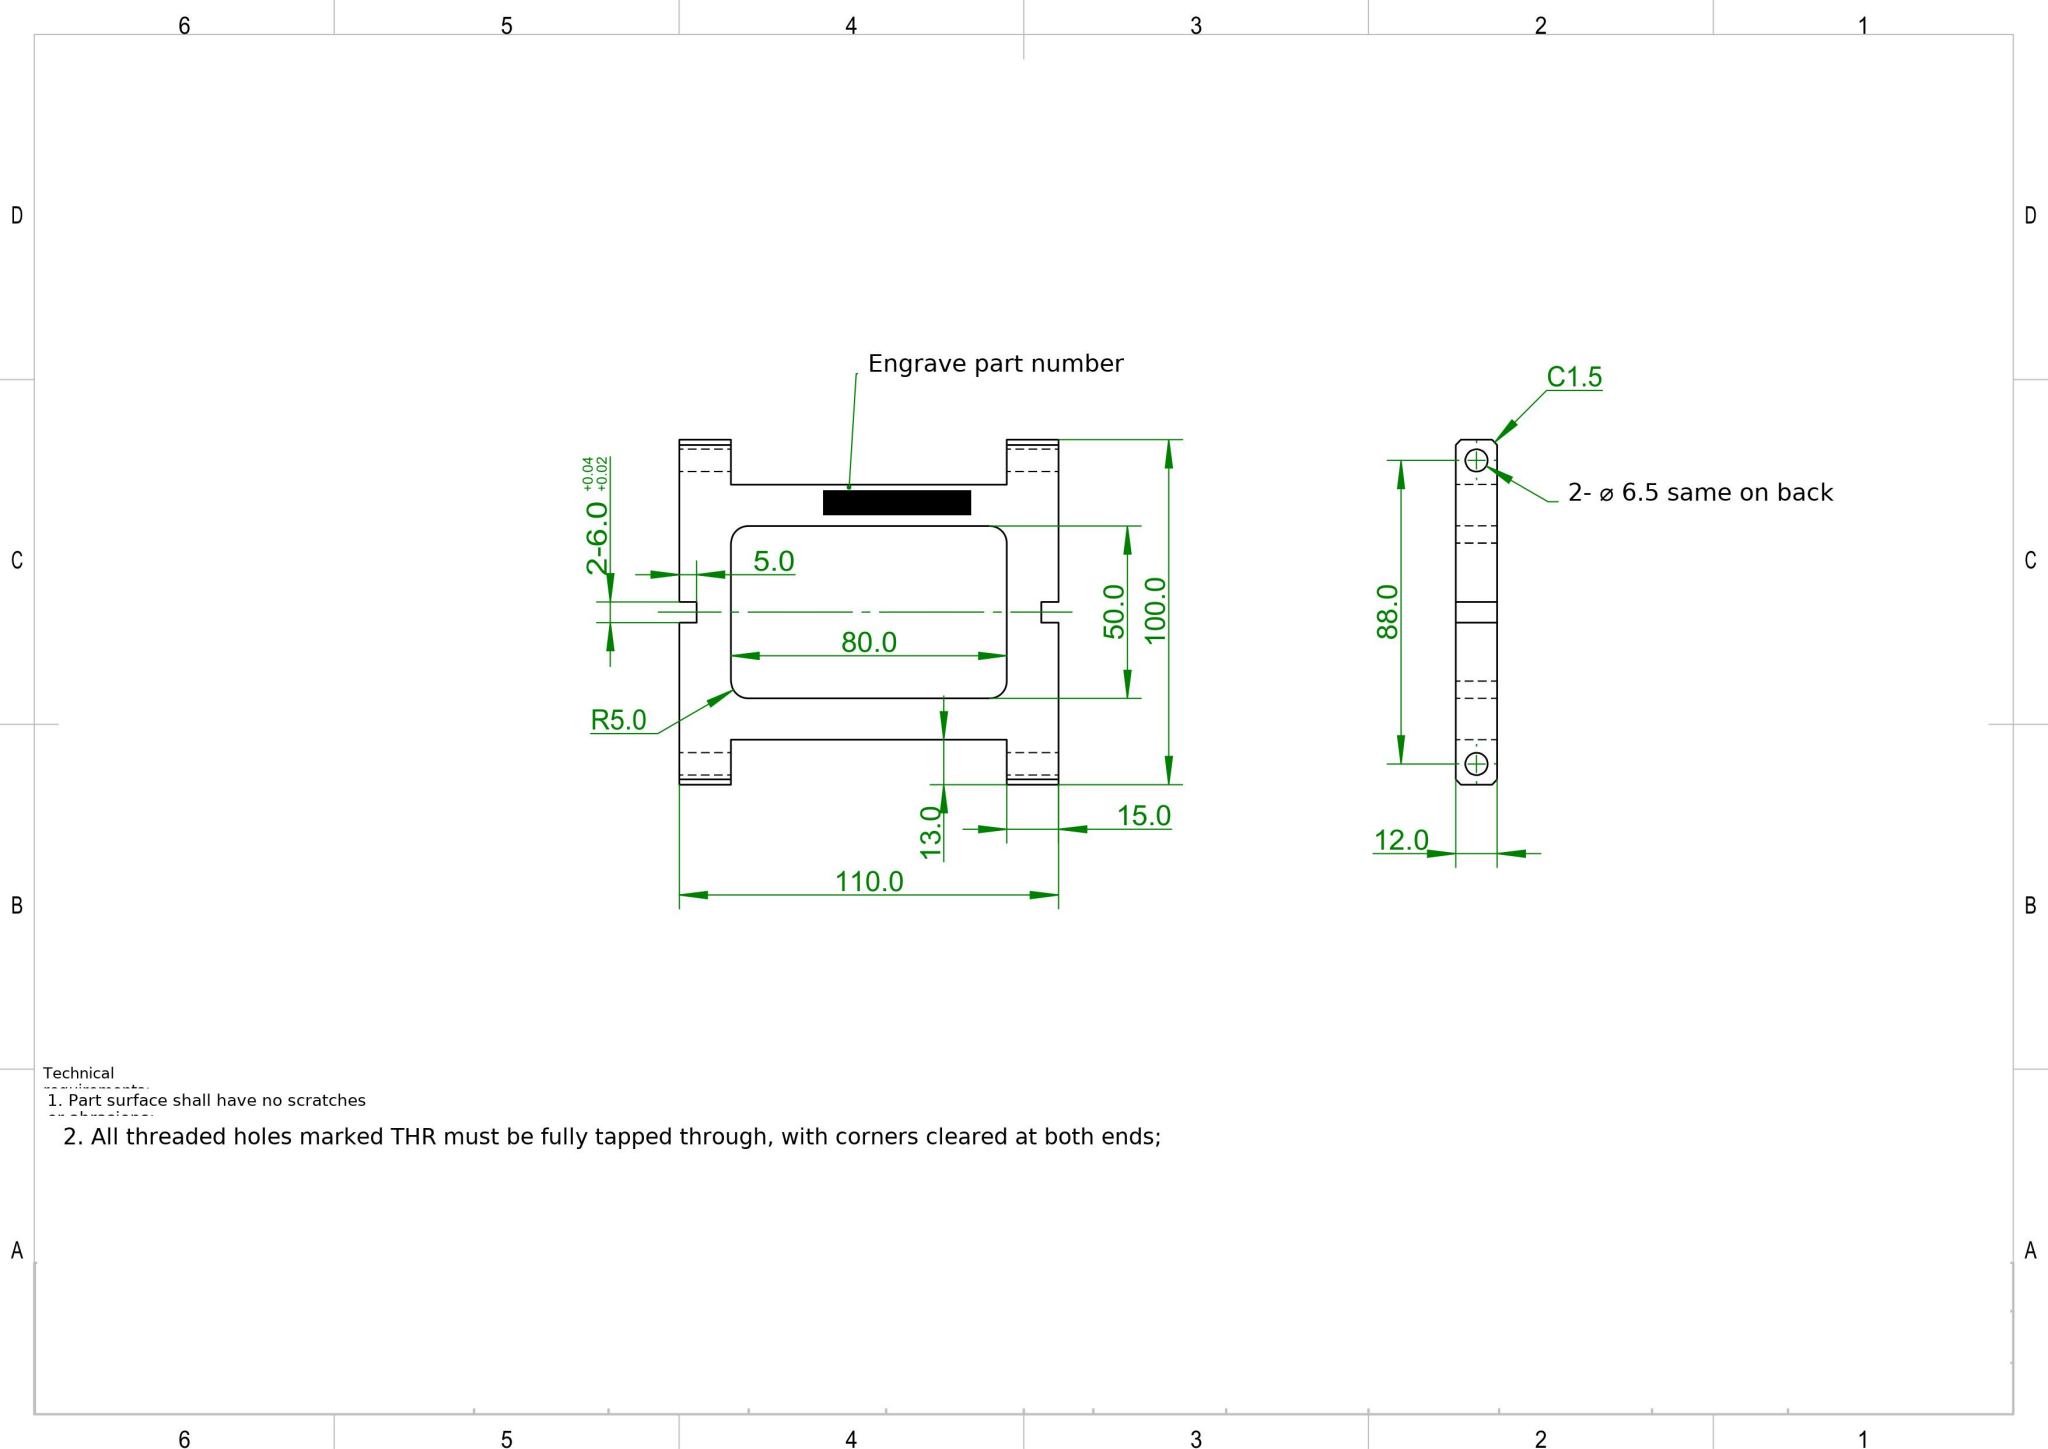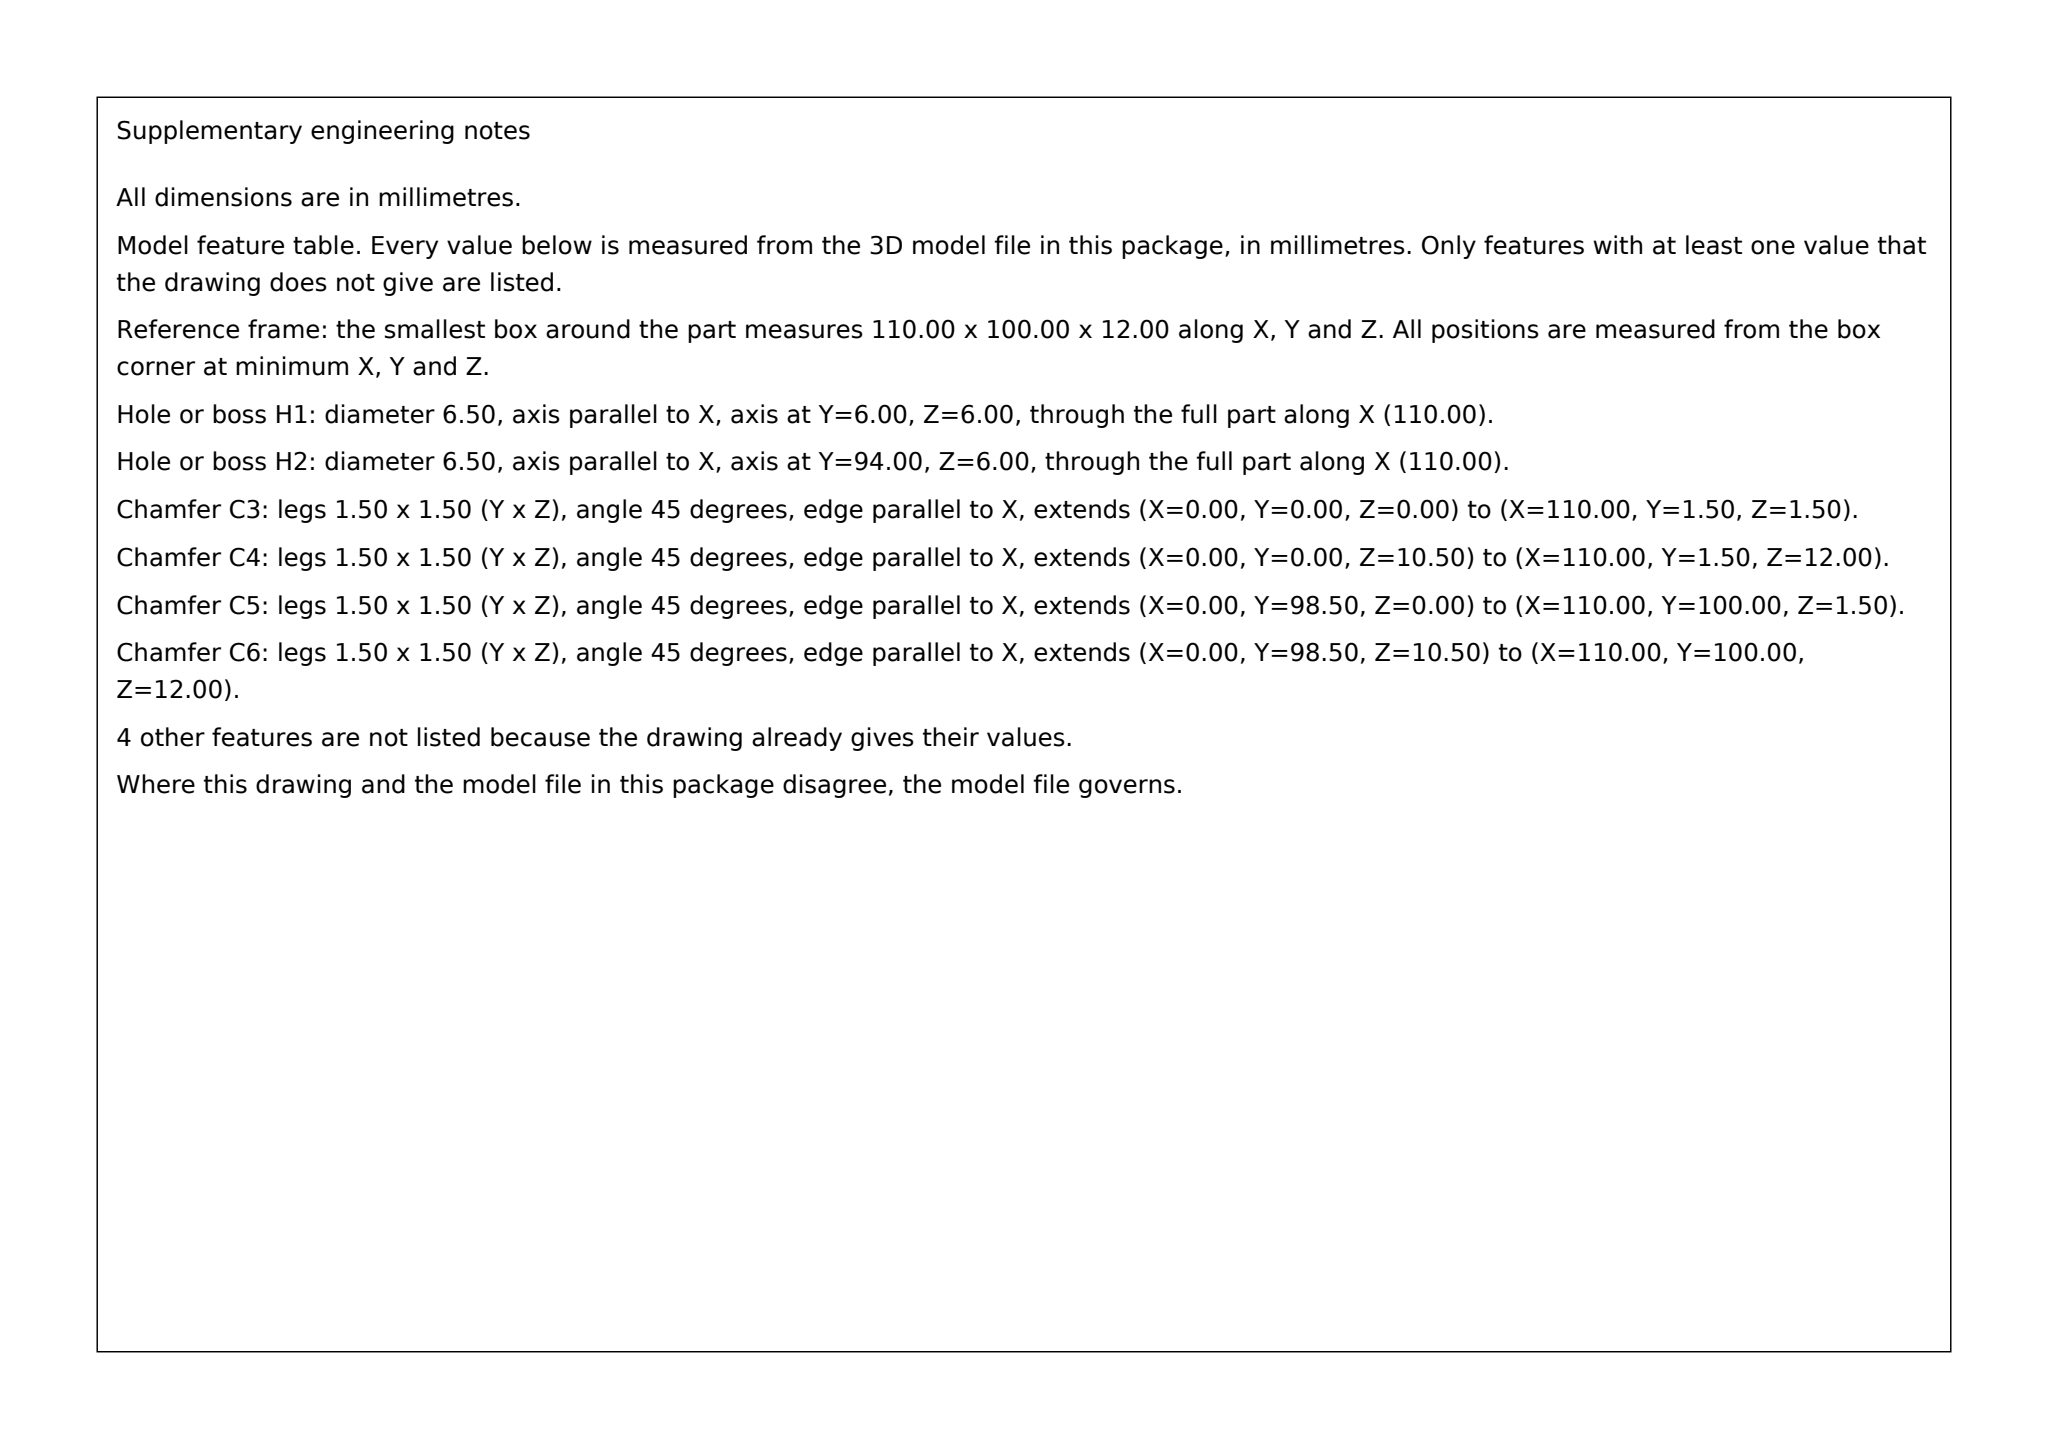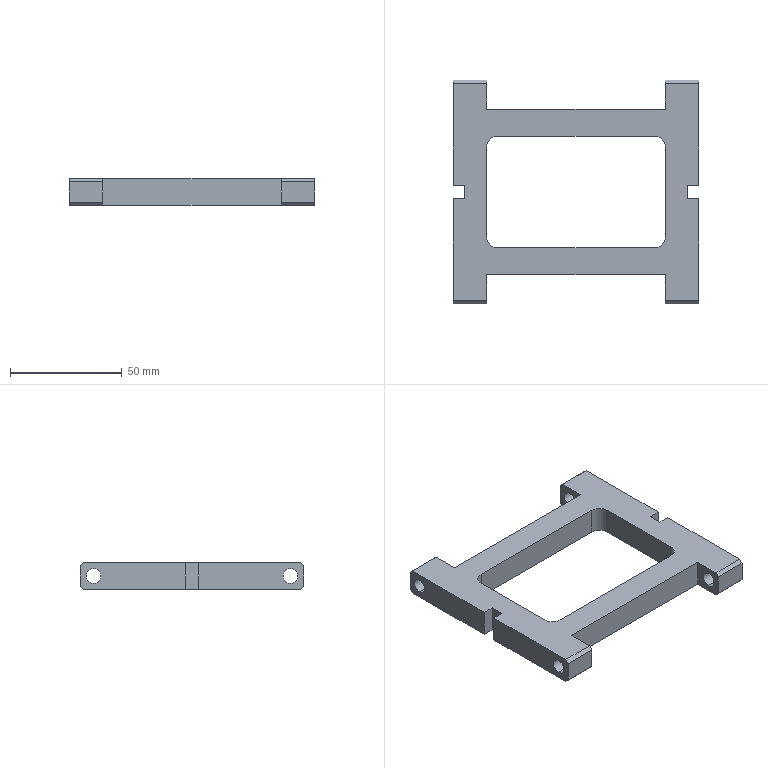Part | SolidWorks | mm | 1 solid | 46 faces | box 110 x 100 x 12 mm | volume 56452 mm3 | plane 34 | cylinder 12 | commonest cylinder face diameters 6.5 x8 10 x4
build123d program:
from build123d import *

# Parameters (mm, degrees)
SKETCH1_W                  = 110
SKETCH1_H                  = 100
BOSS_EXTRUDE1_DEPTH        = 6
SKETCH2_W                  = 12
SKETCH2_H                  = 6
CUT_EXTRUDE1_DEPTH         = 5
SKETCH3_W                  = 80
SKETCH3_H                  = 26
CUT_EXTRUDE2_DEPTH         = 76.293
F_6_5_6_5_DIAMETER_HOLE1_D = 6.5
CUT_EXTRUDE3_DEPTH         = 76.293
CHAMFER1_SIZE              = 1.5


with BuildPart() as part:
    # Sketch1 → Boss-Extrude1 (new, symmetric)
    with BuildSketch(Plane.XY):
        Rectangle(SKETCH1_W, SKETCH1_H)
    extrude(amount=BOSS_EXTRUDE1_DEPTH, both=True)

    # Sketch2 → Cut-Extrude1 (cut)
    with BuildSketch(Plane(origin=(55, 0, 0), x_dir=(0, 0, -1), z_dir=(1, 0, 0))):
        Rectangle(SKETCH2_W, SKETCH2_H)
    cut_extrude1 = extrude(amount=-CUT_EXTRUDE1_DEPTH, mode=Mode.SUBTRACT)

    # Mirror1: Cut-Extrude1 across plane
    add(cut_extrude1.mirror(Plane(origin=(0, 0, 0), x_dir=(0, 0, 1), z_dir=(1, 0, 0))), mode=Mode.SUBTRACT)

    # Sketch3 → Cut-Extrude2 (cut, through all)
    with BuildSketch(Plane.XY.offset(6)):
        with Locations((0, 50)):
            Rectangle(SKETCH3_W, SKETCH3_H)
        with Locations((0, -50)):
            Rectangle(SKETCH3_W, SKETCH3_H)
    extrude(amount=-CUT_EXTRUDE2_DEPTH, mode=Mode.SUBTRACT)

    # 6.5 _6.5_ Diameter Hole1 (through all)
    with Locations(Plane(origin=(55, 0, 0), x_dir=(0, 0, -1), z_dir=(1, 0, 0))):
        with Locations((0, 44), (0, -44)):
            Hole(F_6_5_6_5_DIAMETER_HOLE1_D / 2)

    # Sketch6 → Cut-Extrude3 (cut, through all)
    with BuildSketch(Plane.XY.offset(6)):
        with BuildLine():
            Line((-35, -25), (35, -25))
            ThreePointArc((35, -25), (38.536, -23.536), (40, -20))
            Line((40, -20), (40, 20))
            ThreePointArc((40, 20), (38.536, 23.536), (35, 25))
            Line((35, 25), (-35, 25))
            ThreePointArc((-35, 25), (-38.536, 23.536), (-40, 20))
            Line((-40, 20), (-40, -20))
            ThreePointArc((-40, -20), (-38.536, -23.536), (-35, -25))
        make_face()
    extrude(amount=-CUT_EXTRUDE3_DEPTH, mode=Mode.SUBTRACT)

    # Chamfer1
    chamfer1_edges = [part.edges().sort_by_distance(p)[0] for p in [
        (-47.5, -50, 6),
        (-47.5, -50, -6),
        (-47.5, 50, -6),
        (-47.5, 50, 6),
        (47.5, 50, -6),
        (47.5, -50, -6),
        (47.5, -50, 6),
        (47.5, 50, 6),
    ]]
    chamfer(chamfer1_edges, length=CHAMFER1_SIZE)


solid = part.part